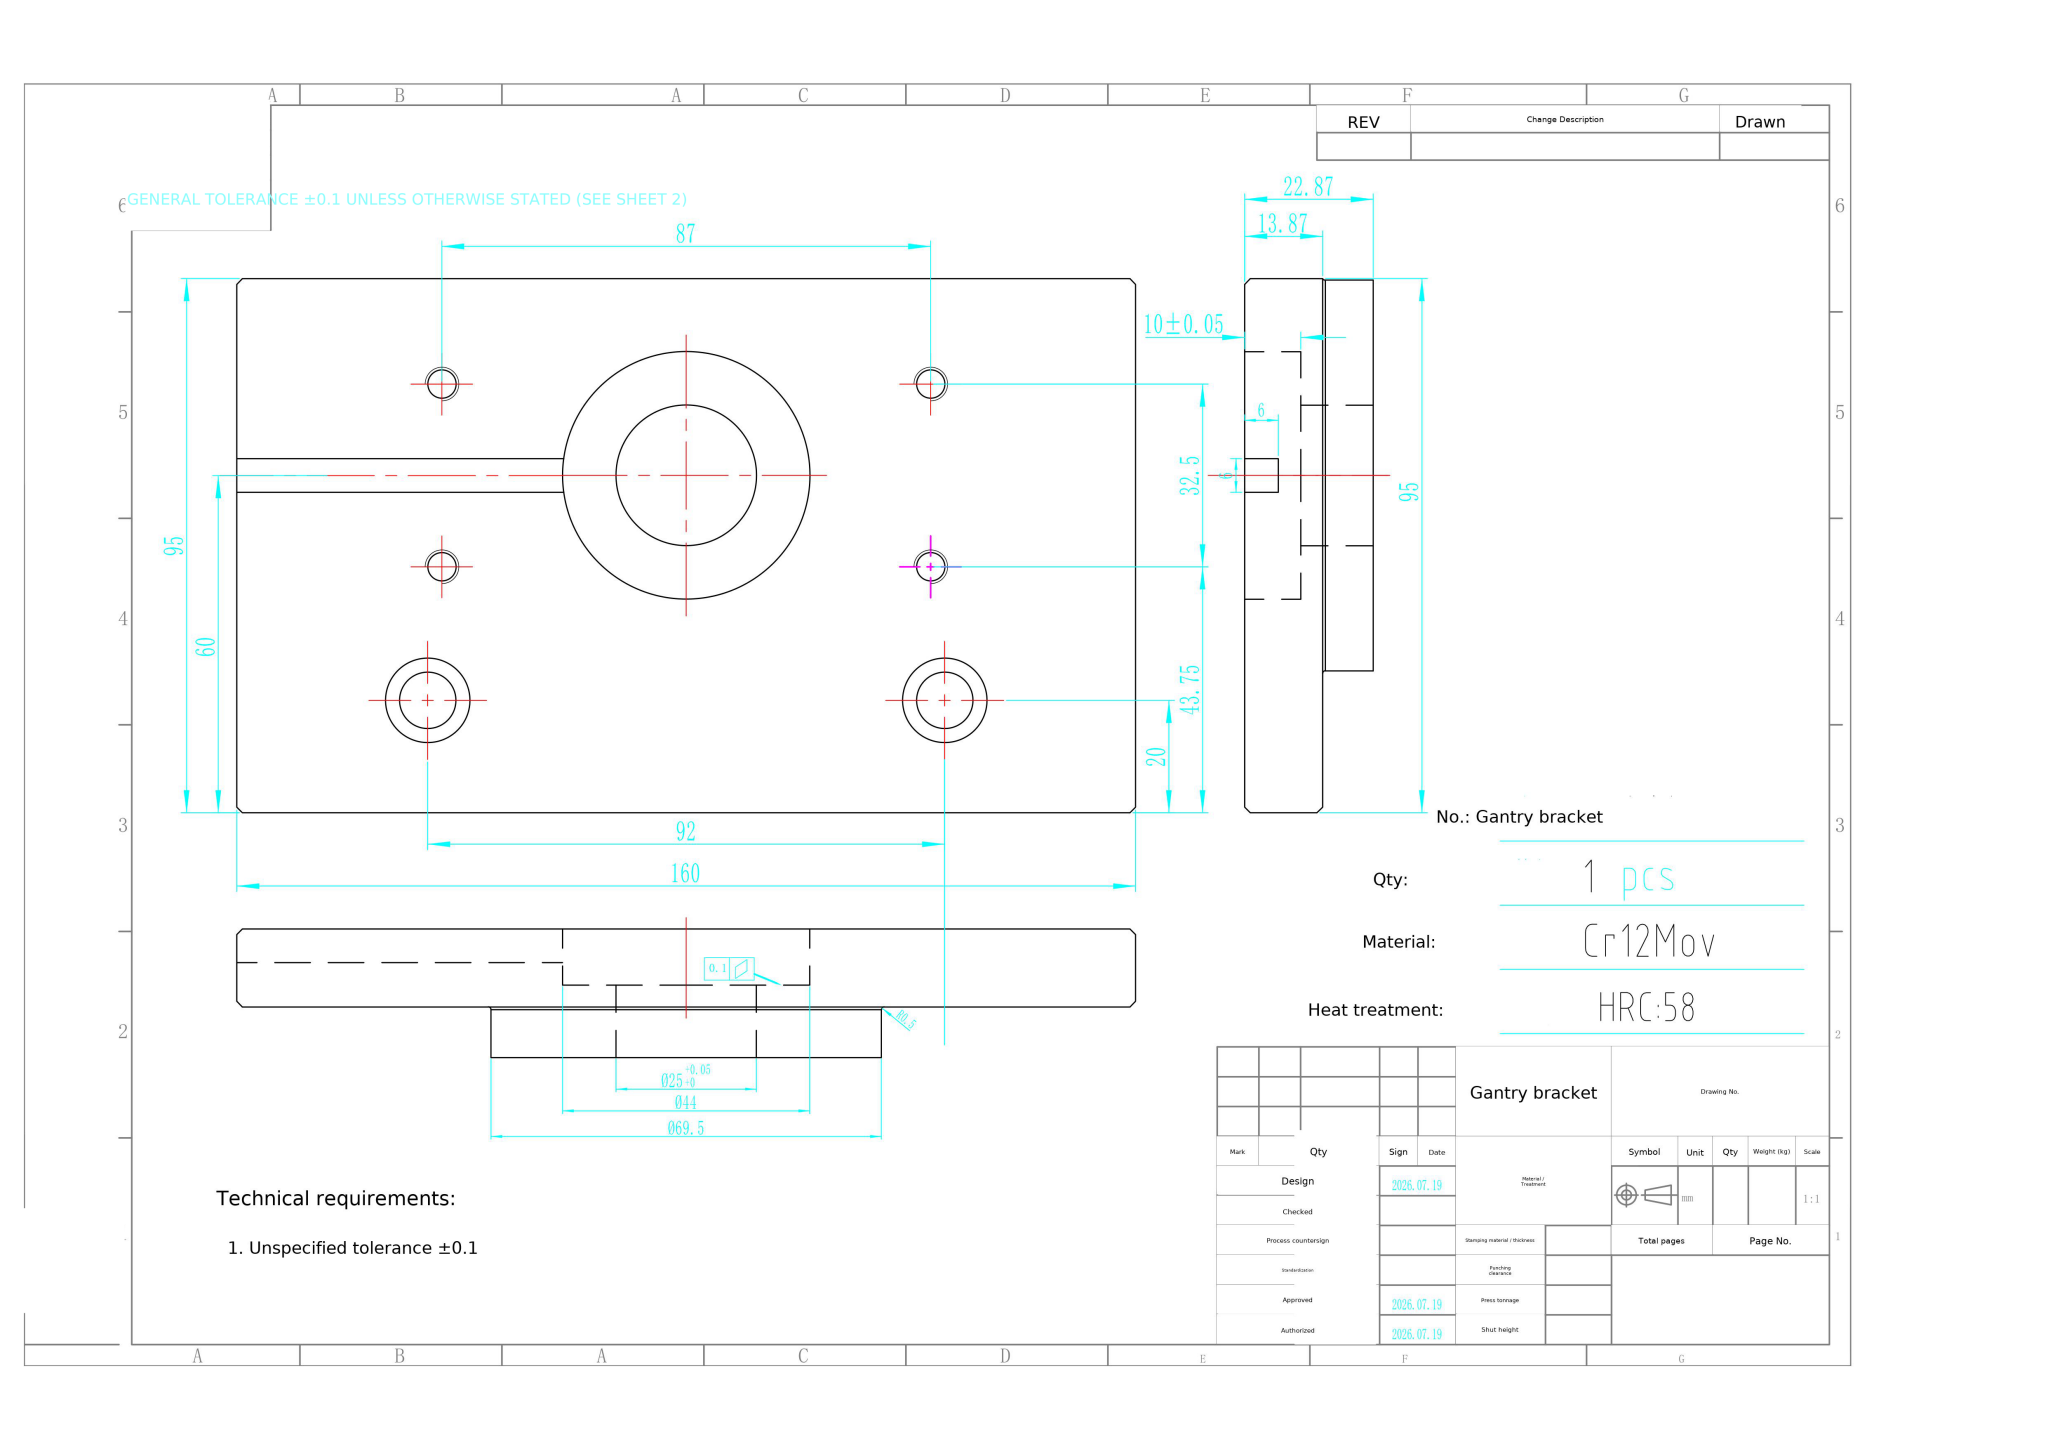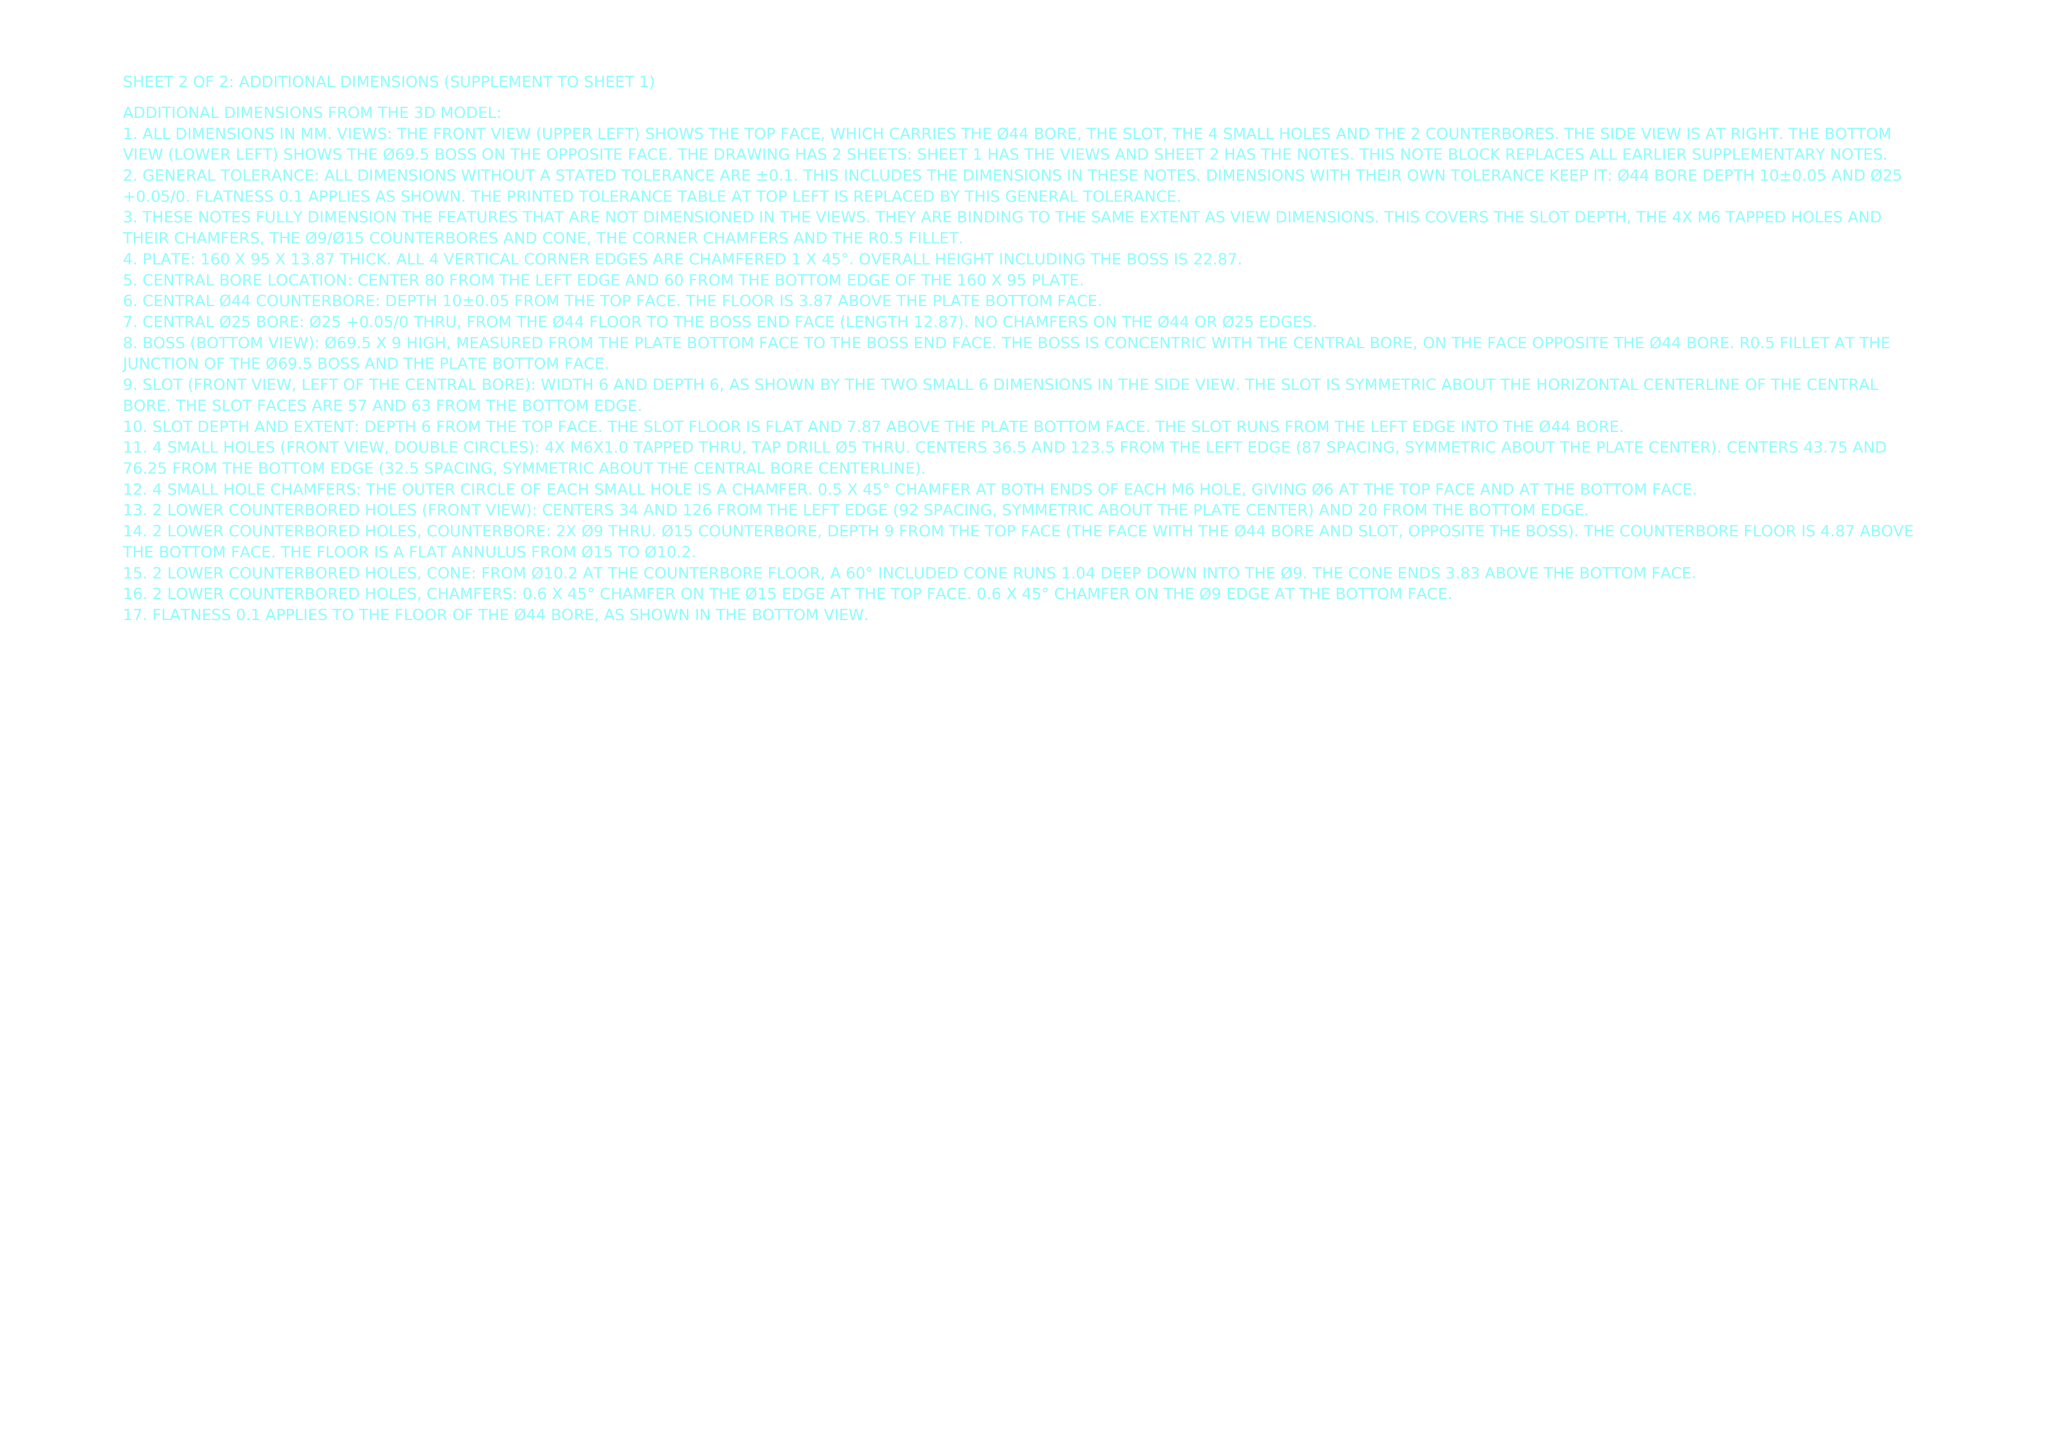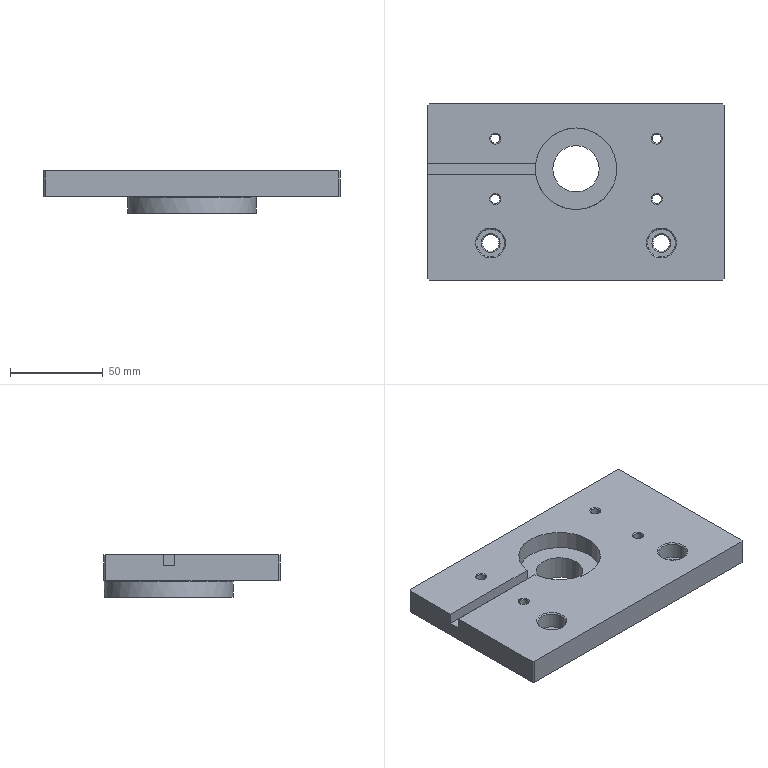Part | NX | mm | 1 solid | 44 faces | box 160 x 95 x 22.87 mm | volume 216385 mm3 | plane 17 | cone 14 | cylinder 11 | torus 1 | spline 1 | commonest cylinder face diameters 5 x4 9 x2 15 x2 25 x1 44 x1 69.5 x1